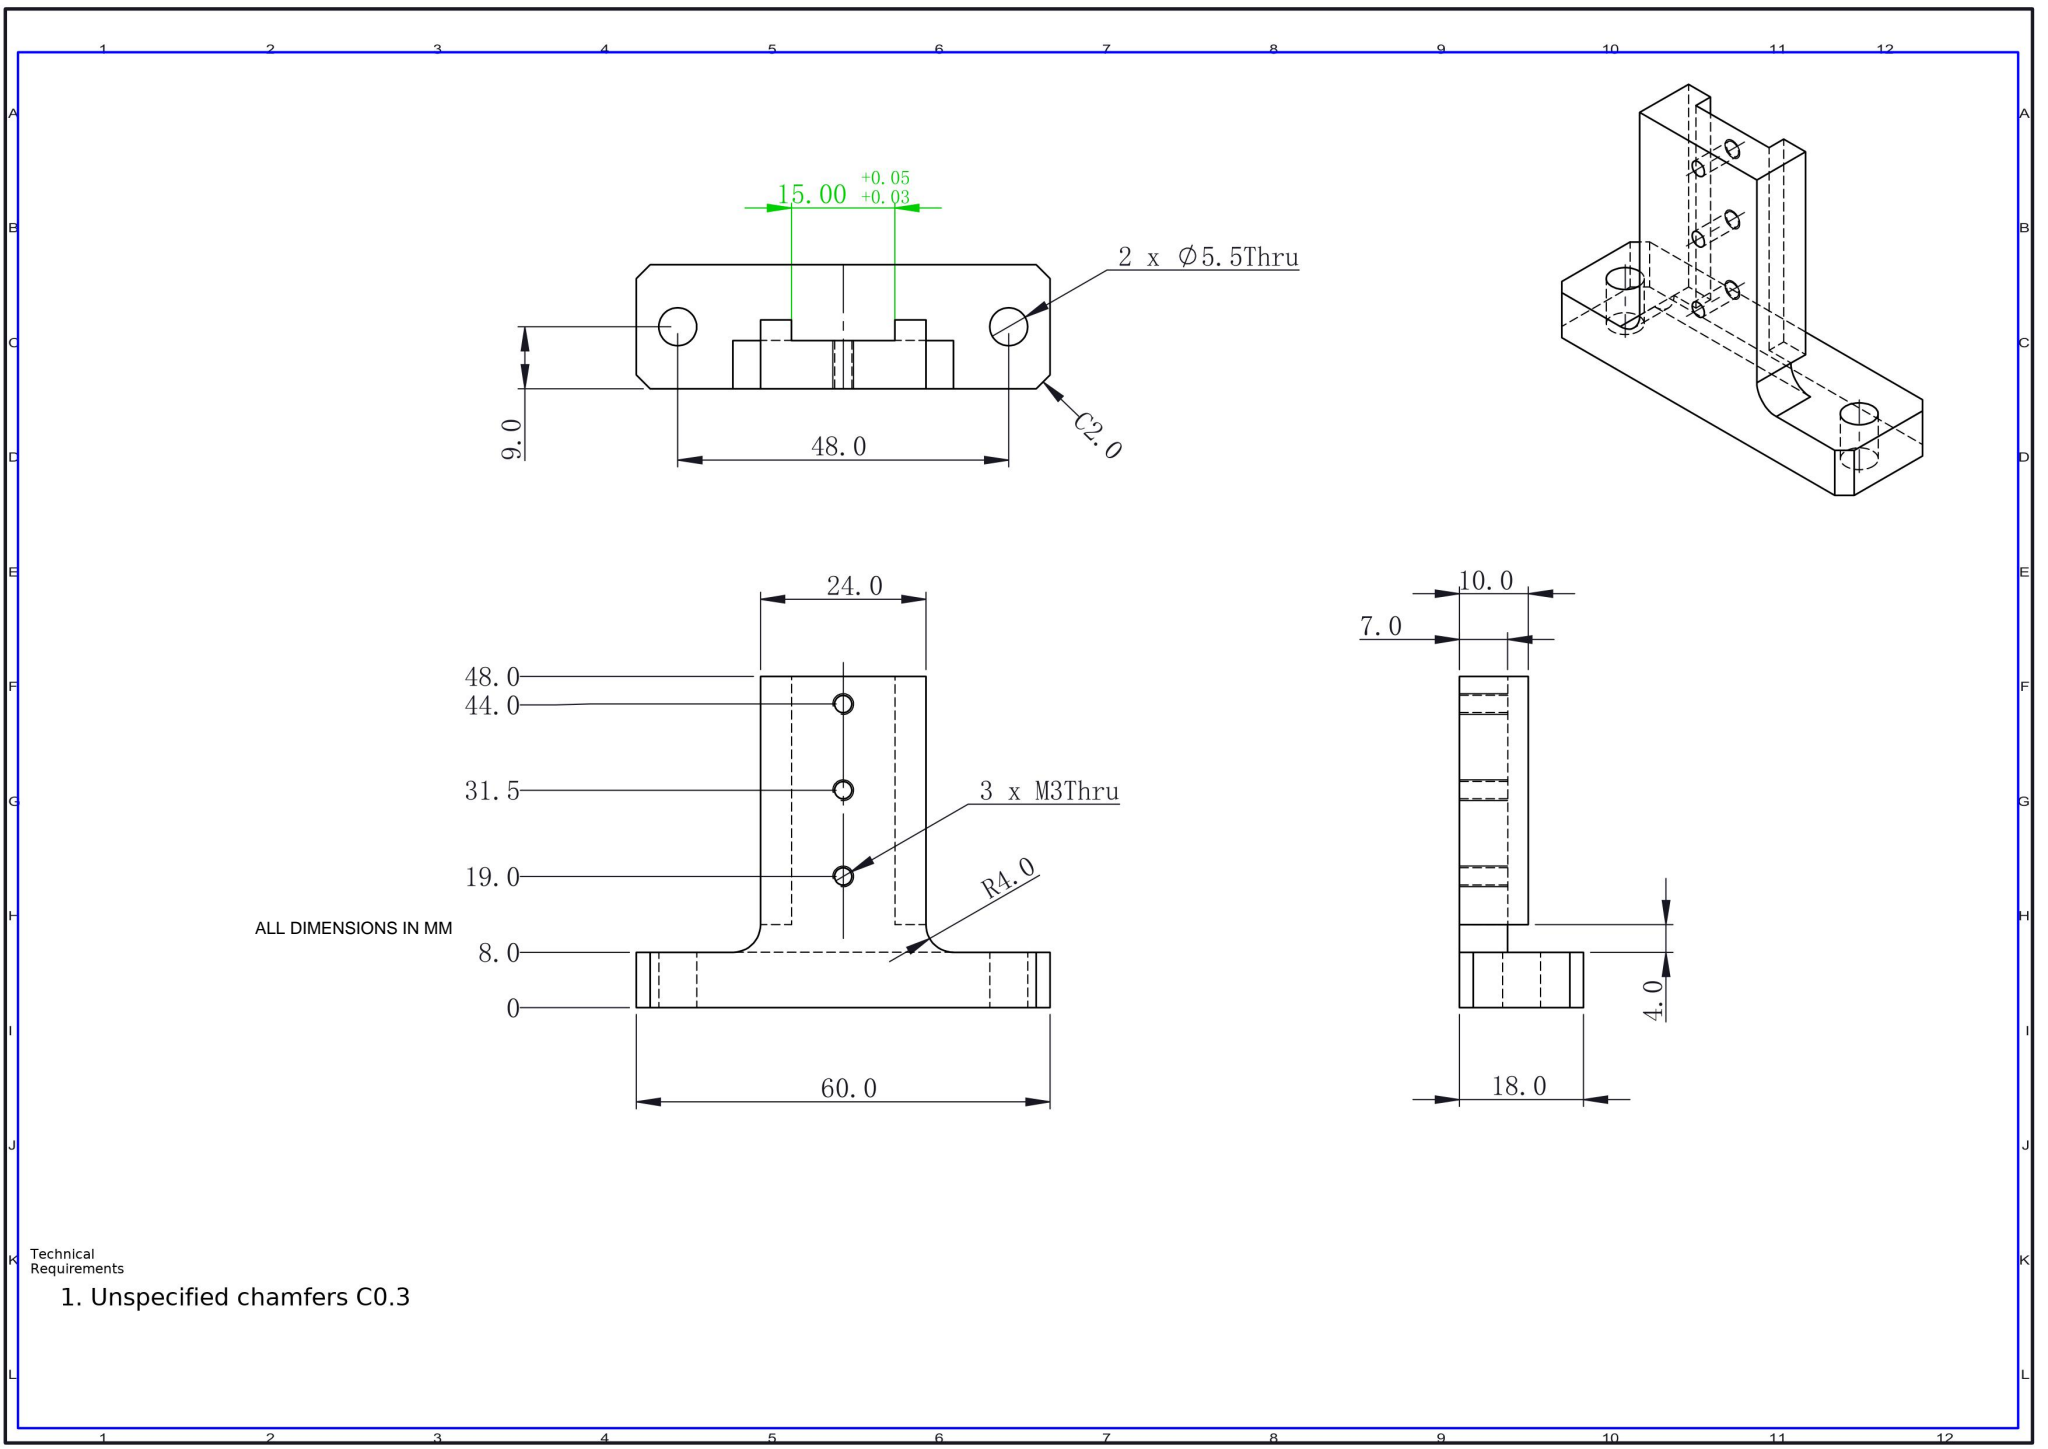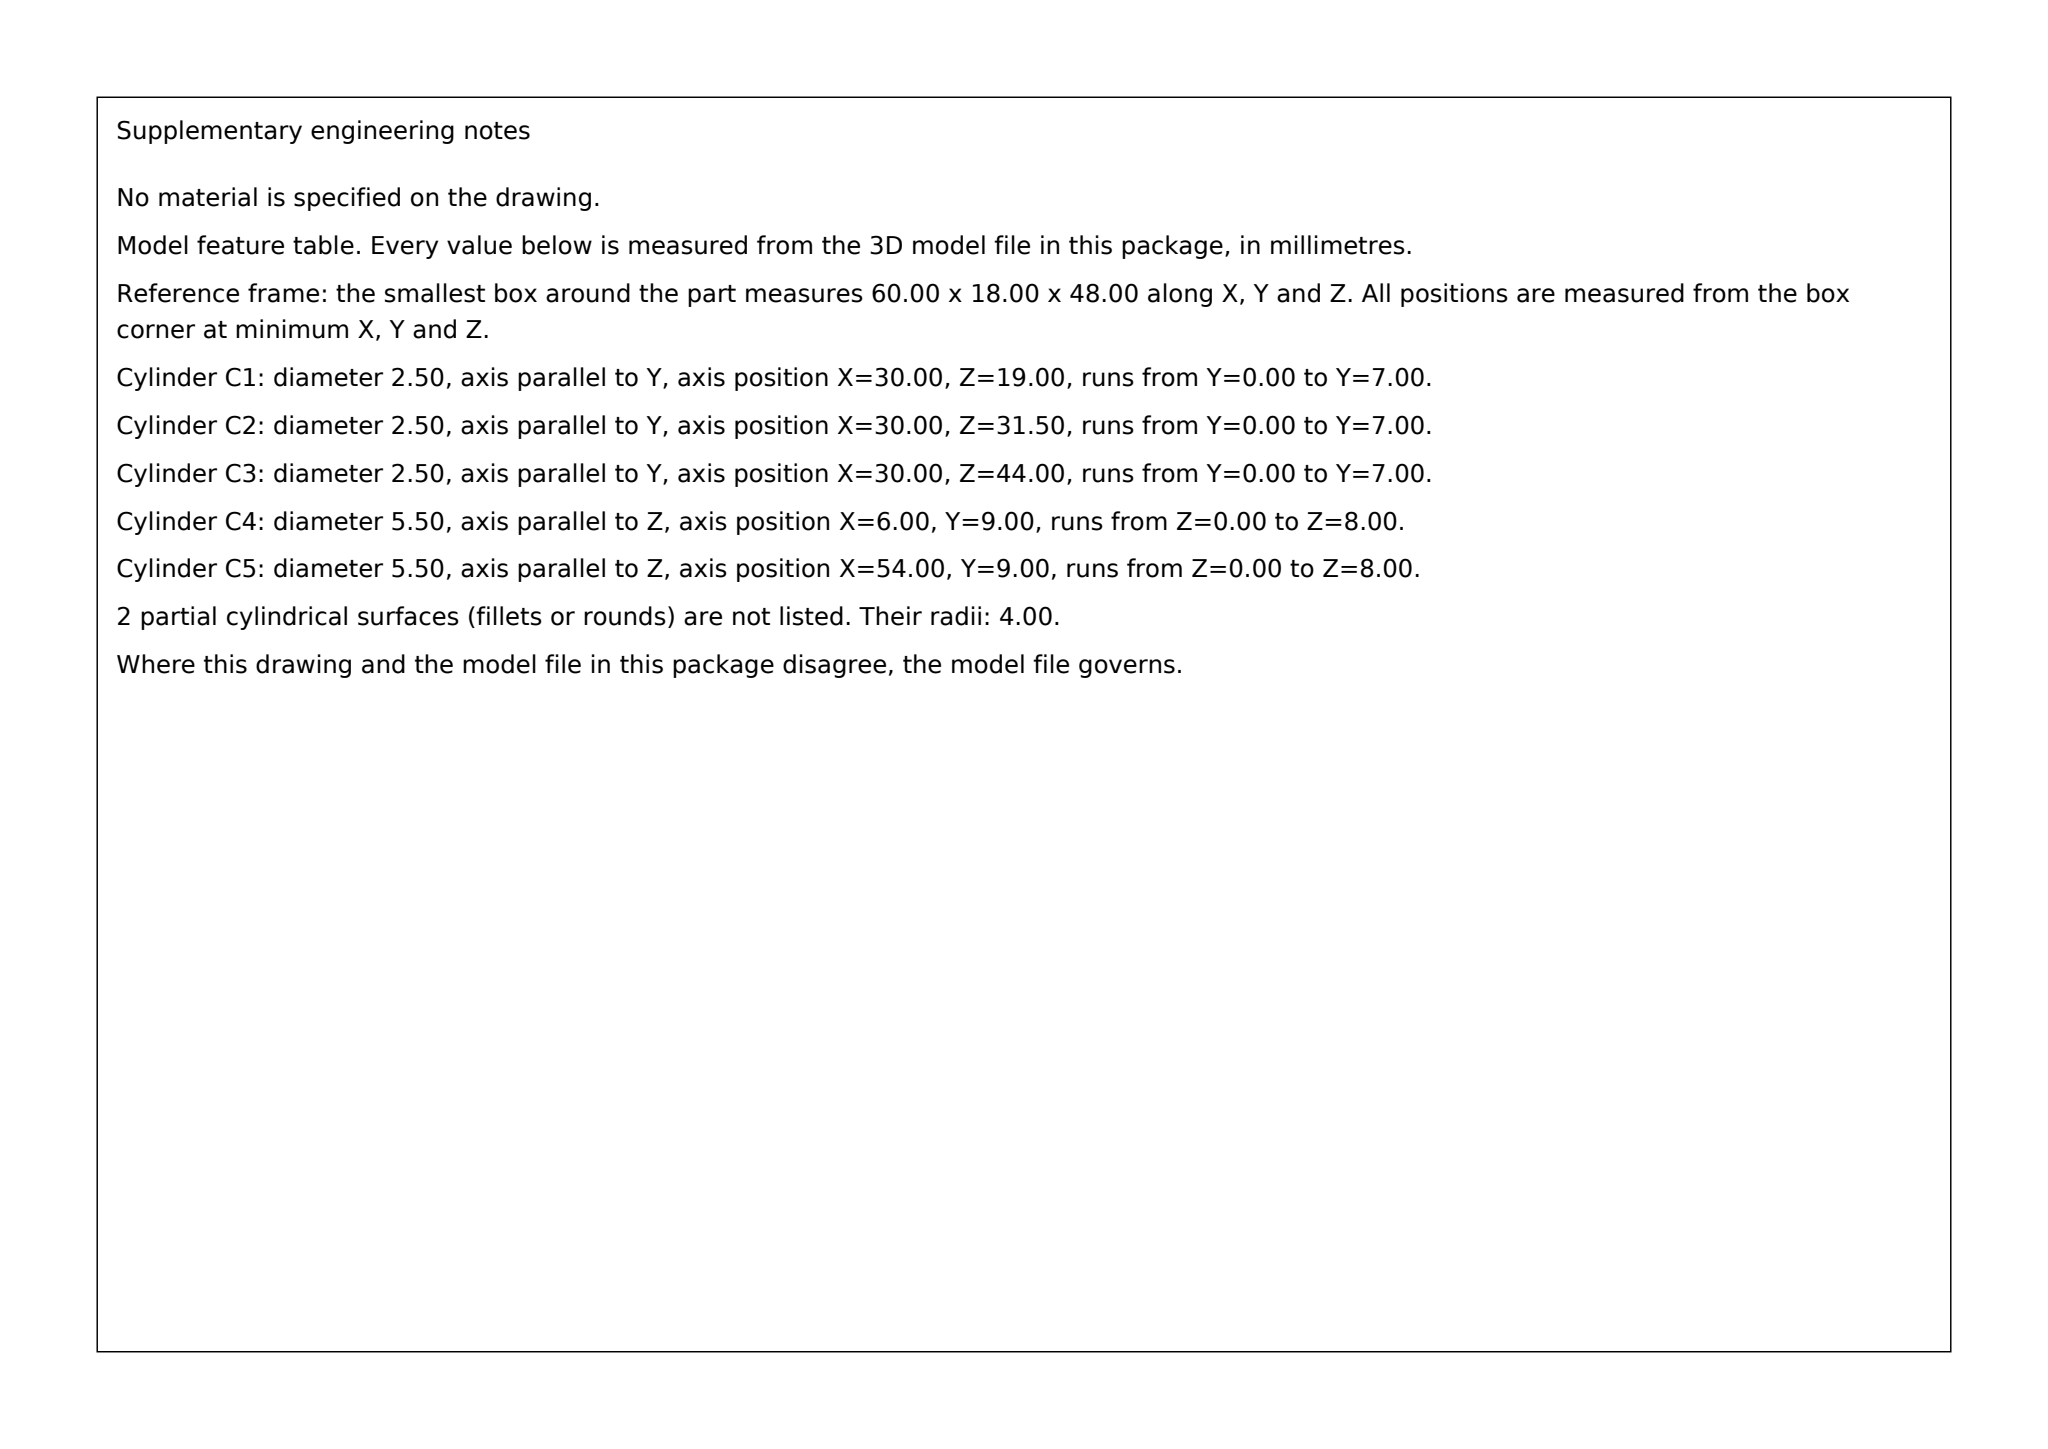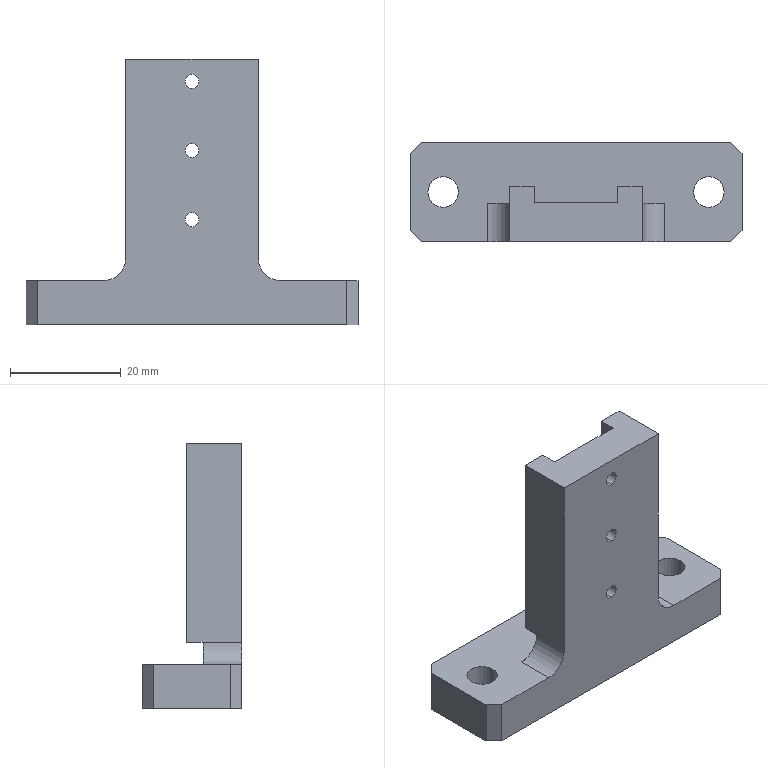Part | SolidWorks | mm | 1 solid | 32 faces | box 60 x 18 x 48 mm | volume 15833 mm3 | plane 20 | cylinder 12 | commonest cylinder face diameters 2.5 x6 5.5 x4 8 x2
build123d program:
from build123d import *

# Parameters (mm, degrees)
SKETCH1_W            = 60
SKETCH1_H            = 18
BOSS_EXTRUDE1_DEPTH  = 8
SKETCH2_W            = 24
SKETCH2_H            = 10
BOSS_EXTRUDE2_DEPTH  = 40
SKETCH3_W            = 15
SKETCH3_H            = 40
CUT_EXTRUDE1_DEPTH   = 3
SKETCH4_W            = 24
SKETCH4_H            = 4
CUT_EXTRUDE5_DEPTH   = 58.663
FILLET1_R            = 4
M4_CLEARANCE_HOLE1_D = 5.5
M3_TAPPED_HOLE1_D    = 2.5
CHAMFER1_SIZE        = 2


with BuildPart() as part:
    # Sketch1 → Boss-Extrude1 (new body)
    with BuildSketch(Plane.XY):
        Rectangle(SKETCH1_W, SKETCH1_H)
    extrude(amount=BOSS_EXTRUDE1_DEPTH)

    # Sketch2 → Boss-Extrude2 (add)
    with BuildSketch(Plane.XY.offset(8)):
        with Locations((0, -4)):
            Rectangle(SKETCH2_W, SKETCH2_H)
    extrude(amount=BOSS_EXTRUDE2_DEPTH)

    # Sketch3 → Cut-Extrude1 (cut)
    with BuildSketch(Plane(origin=(0, 1, 0), x_dir=(1, 0, 0), z_dir=(0, 1, 0))):
        with Locations((0, -28)):
            Rectangle(SKETCH3_W, SKETCH3_H)
    extrude(amount=-CUT_EXTRUDE1_DEPTH, mode=Mode.SUBTRACT)

    # Sketch4 → Cut-Extrude5 (cut, through all)
    with BuildSketch(Plane(origin=(0, -2, 0), x_dir=(1, 0, 0), z_dir=(0, 1, 0))):
        with Locations((0, -10)):
            Rectangle(SKETCH4_W, SKETCH4_H)
    extrude(amount=CUT_EXTRUDE5_DEPTH, mode=Mode.SUBTRACT)

    # Fillet1
    fillet1_edges = [part.edges().sort_by_distance(p)[0] for p in [
        (12, -5.5, 8),
        (-12, -5.5, 8),
    ]]
    fillet(fillet1_edges, radius=FILLET1_R)

    # M4 Clearance Hole1 (through all)
    with Locations(Plane.XY.offset(8)):
        with Locations((24, 0), (-24, 0)):
            Hole(M4_CLEARANCE_HOLE1_D / 2)

    # M3 Tapped Hole1 (through all)
    with Locations(Plane(origin=(0, -2, 0), x_dir=(1, 0, 0), z_dir=(0, 1, 0))):
        with Locations((0, -19), (0, -31.5), (0, -44)):
            Hole(M3_TAPPED_HOLE1_D / 2)

    # Chamfer1
    chamfer1_edges = [part.edges().sort_by_distance(p)[0] for p in [
        (30, -9, 4),
        (-30, -9, 4),
        (-30, 9, 4),
        (30, 9, 4),
    ]]
    chamfer(chamfer1_edges, length=CHAMFER1_SIZE)


solid = part.part